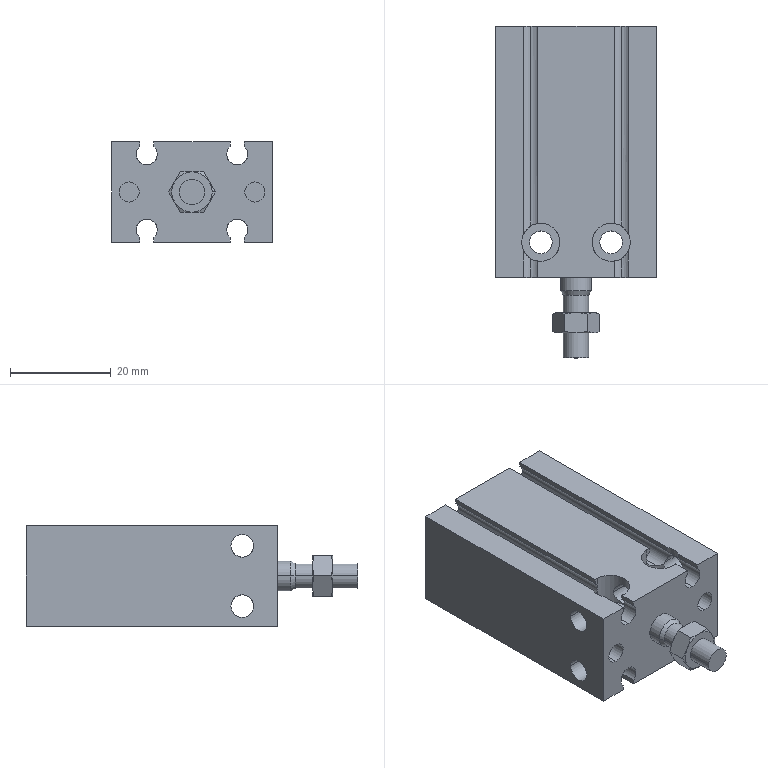Component | SolidWorks | CDUSeriesCylinder-1 | 2 solids | 123 faces | box 32 x 66 x 20 mm | volume 27113 mm3 | cylinder 62 | plane 45 | cone 16 | commonest cylinder face diameters 7.6 x20 4.5 x16 5 x8 4 x8 4.2 x8 6 x2